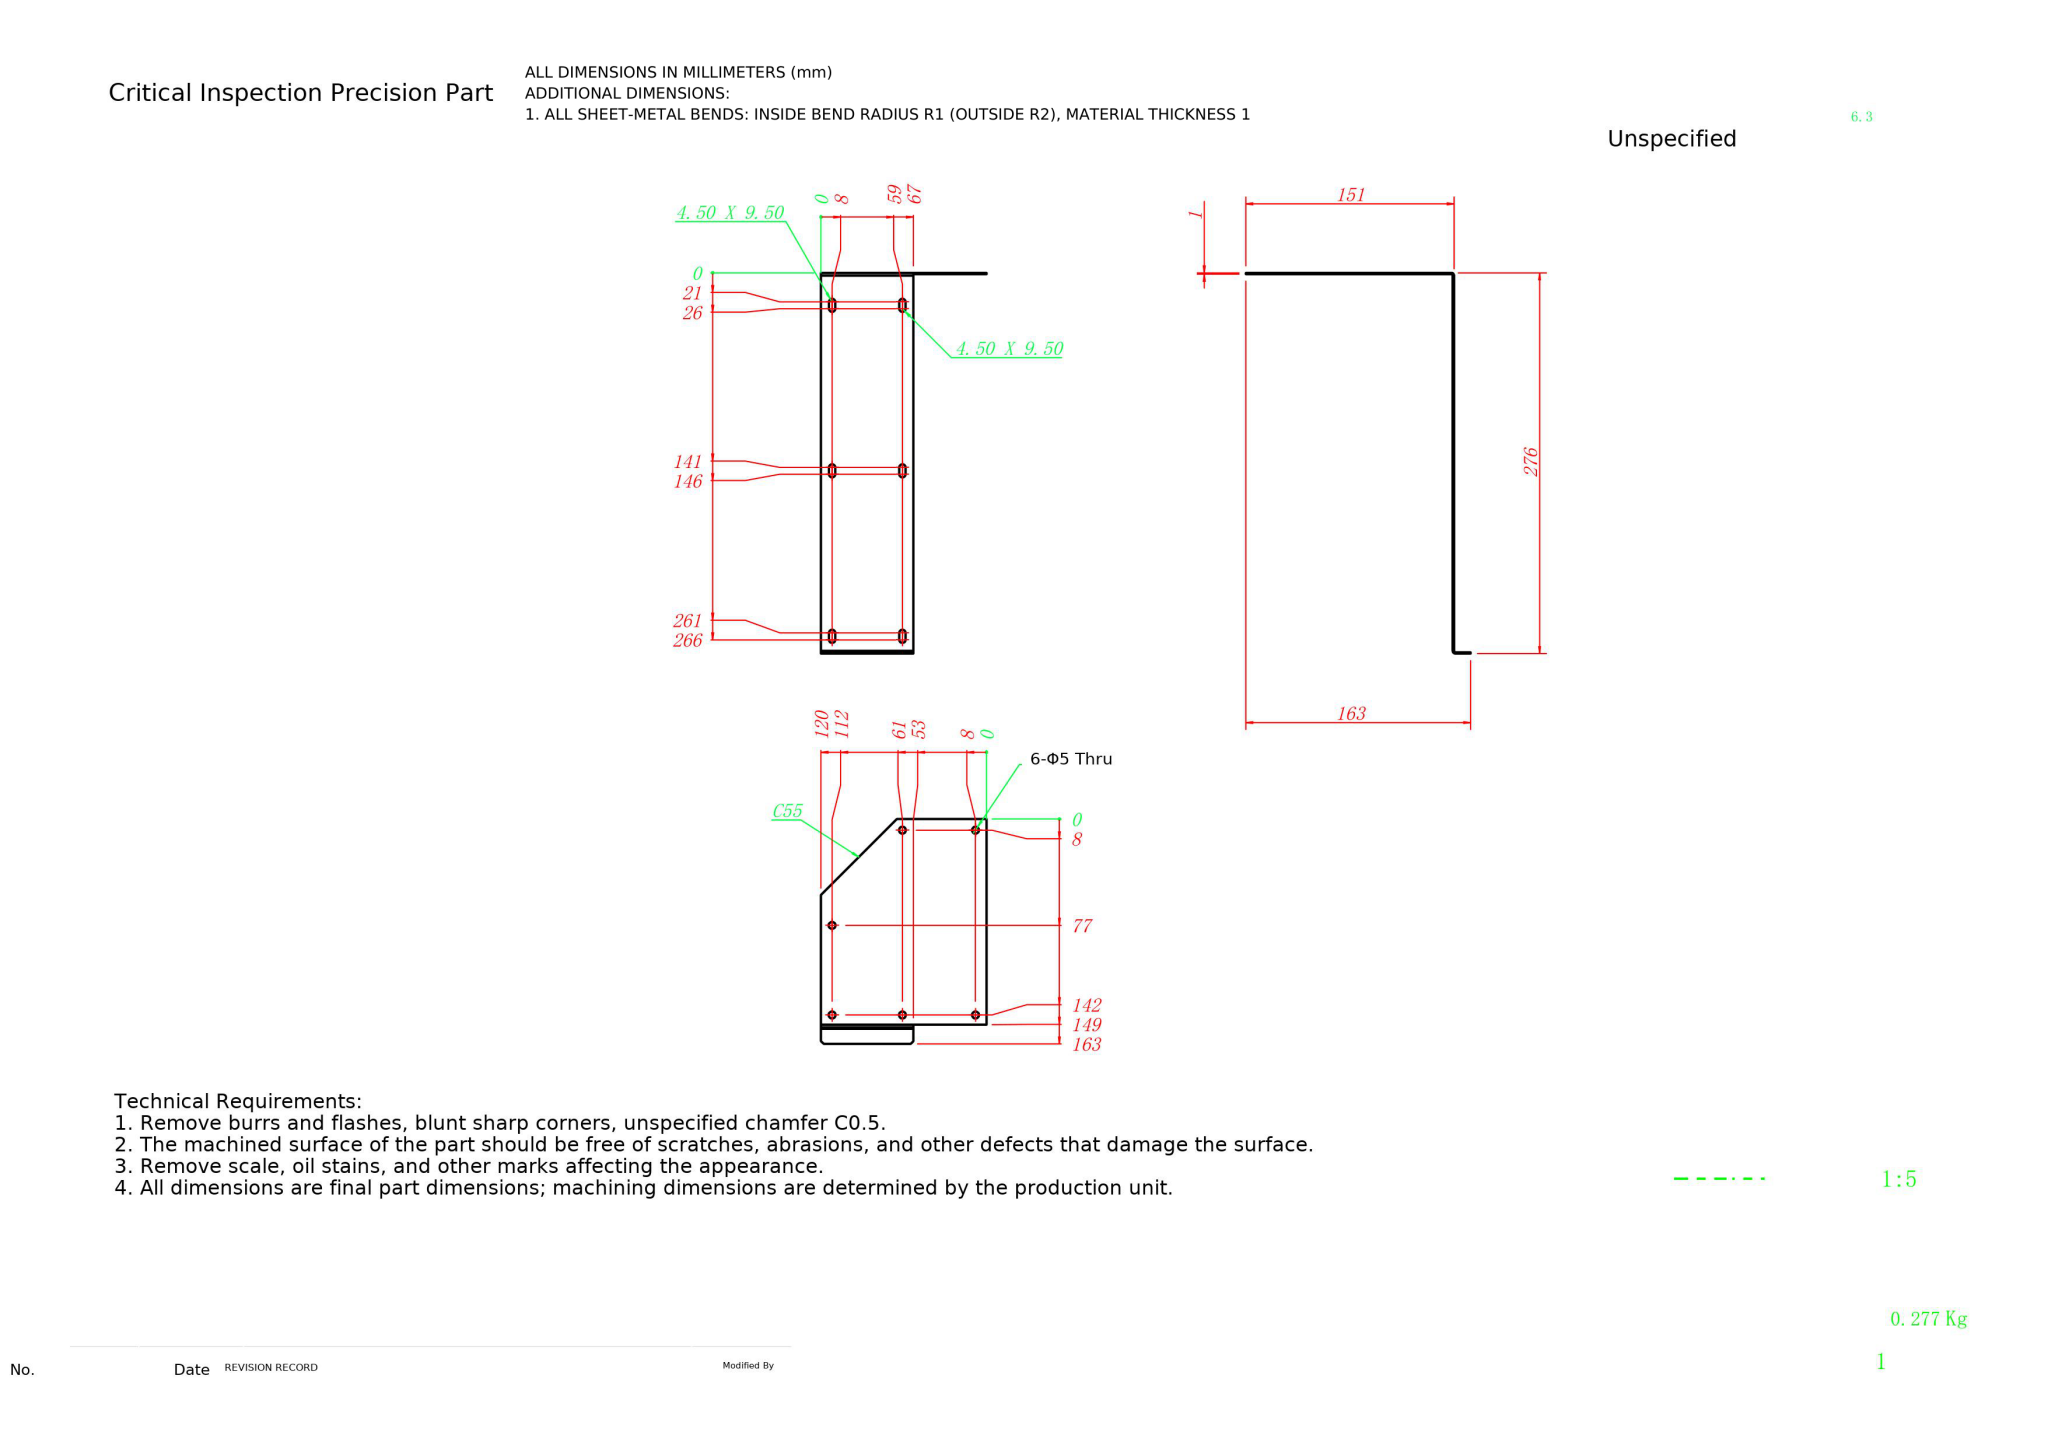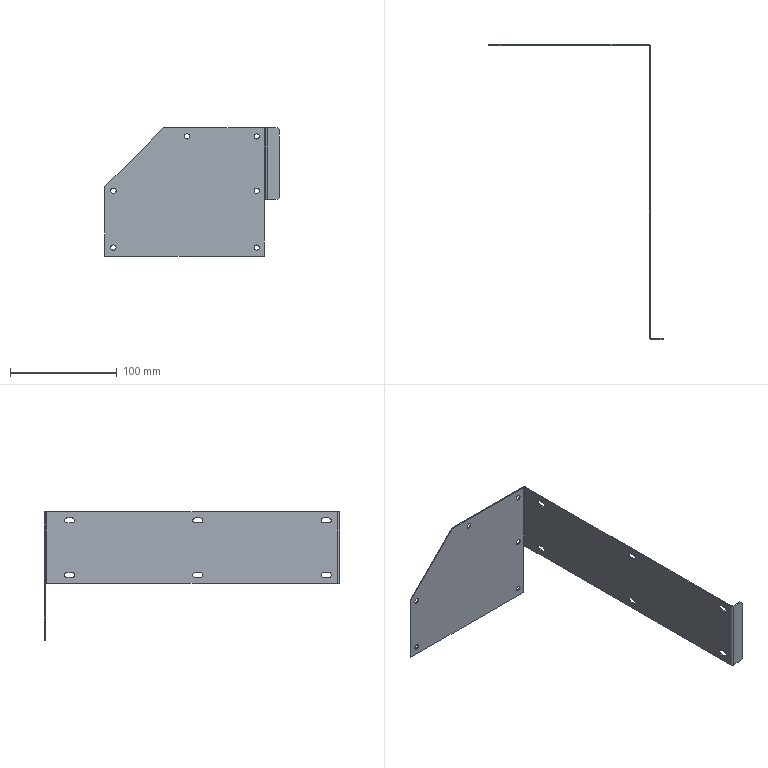Part | NX | mm | 1 solid | 55 faces | box 163 x 276 x 120 mm | volume 35292 mm3 | cylinder 28 | plane 27 | commonest cylinder face diameters 5 x12 4.5 x12 2 x2 4 x2